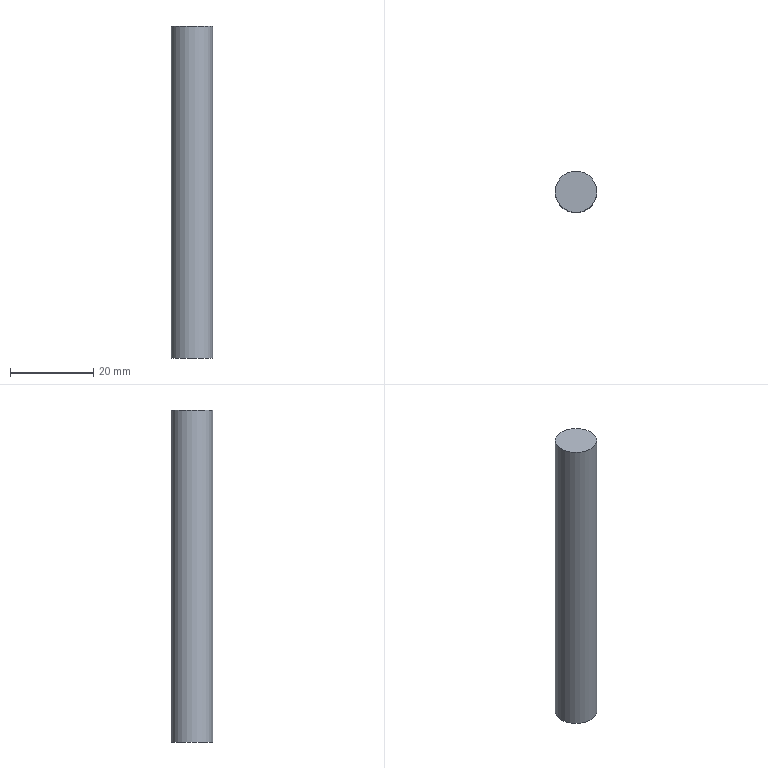Component | NX | FIXING_SCREW | 1 solid | 3 faces | box 10 x 10 x 80 mm | volume 6283 mm3 | plane 2 | cylinder 1 | commonest cylinder face diameters 10 x1
STEP:
#1=CARTESIAN_POINT('',(0.,0.,0.));
#2=DIRECTION('',(0.,0.,1.));
#3=DIRECTION('',(1.,0.,0.));
#4=AXIS2_PLACEMENT_3D('',#1,#2,#3);
#5=CARTESIAN_POINT('',(-5.,93.,139.));
#6=VERTEX_POINT('',#5);
#7=CARTESIAN_POINT('',(-0.,93.,139.));
#8=DIRECTION('',(0.,0.,-1.));
#9=DIRECTION('',(-1.,0.,0.));
#10=AXIS2_PLACEMENT_3D('',#7,#8,#9);
#11=CIRCLE('',#10,5.);
#12=CARTESIAN_POINT('',(-0.,93.,139.));
#13=DIRECTION('',(0.,0.,1.));
#14=DIRECTION('',(-1.,0.,0.));
#15=AXIS2_PLACEMENT_3D('',#12,#13,#14);
#16=PLANE('',#15);
#17=CARTESIAN_POINT('',(5.,0.));
#18=CARTESIAN_POINT('',(5.,-8.66));
#19=CARTESIAN_POINT('',(-2.5,-4.33));
#20=CARTESIAN_POINT('',(-10.,-0.));
#21=CARTESIAN_POINT('',(-2.5,4.33));
#22=CARTESIAN_POINT('',(5.,8.66));
#23=CARTESIAN_POINT('',(5.,0.));
#24=(BOUNDED_CURVE()B_SPLINE_CURVE(2,(#17,#18,#19,#20,#21,#22,#23),.UNSPECIFIED.,.T.,.F.)B_SPLINE_CURVE_WITH_KNOTS((1,2,2,2,2,1),(-2.094,0.,2.094,4.189,6.283,8.378),.UNSPECIFIED.)CURVE()GEOMETRIC_REPRESENTATION_ITEM()RATIONAL_B_SPLINE_CURVE((1.,0.5,1.,0.5,1.,0.5,1.))REPRESENTATION_ITEM(''));
#25=(GEOMETRIC_REPRESENTATION_CONTEXT(2)PARAMETRIC_REPRESENTATION_CONTEXT()REPRESENTATION_CONTEXT('',''));
#26=DEFINITIONAL_REPRESENTATION('',(#24),#25);
#27=PCURVE('',#16,#26);
#28=CARTESIAN_POINT('',(-0.,93.,59.));
#29=DIRECTION('',(0.,0.,1.));
#30=DIRECTION('',(-1.,0.,0.));
#31=AXIS2_PLACEMENT_3D('',#28,#29,#30);
#32=CYLINDRICAL_SURFACE('',#31,5.);
#33=CARTESIAN_POINT('',(6.283,80.));
#34=DIRECTION('',(-1.,0.));
#35=VECTOR('',#34,1.);
#36=LINE('',#33,#35);
#37=(GEOMETRIC_REPRESENTATION_CONTEXT(2)PARAMETRIC_REPRESENTATION_CONTEXT()REPRESENTATION_CONTEXT('',''));
#38=DEFINITIONAL_REPRESENTATION('',(#36),#37);
#39=PCURVE('',#32,#38);
#40=SURFACE_CURVE('',#11,(#27,#39),.PCURVE_S1.);
#41=EDGE_CURVE('',#6,#6,#40,.T.);
#42=ORIENTED_EDGE('',*,*,#41,.F.);
#43=EDGE_LOOP('',(#42));
#44=FACE_BOUND('',#43,.T.);
#45=ADVANCED_FACE('',(#44),#16,.T.);
#46=CARTESIAN_POINT('',(-5.,93.,59.));
#47=VERTEX_POINT('',#46);
#48=CARTESIAN_POINT('',(-0.,93.,59.));
#49=DIRECTION('',(0.,0.,1.));
#50=DIRECTION('',(-1.,0.,0.));
#51=AXIS2_PLACEMENT_3D('',#48,#49,#50);
#52=CIRCLE('',#51,5.);
#53=CARTESIAN_POINT('',(-0.,93.,59.));
#54=DIRECTION('',(0.,0.,-1.));
#55=DIRECTION('',(1.,0.,0.));
#56=AXIS2_PLACEMENT_3D('',#53,#54,#55);
#57=PLANE('',#56);
#58=CARTESIAN_POINT('',(-5.,0.));
#59=CARTESIAN_POINT('',(-5.,8.66));
#60=CARTESIAN_POINT('',(2.5,4.33));
#61=CARTESIAN_POINT('',(10.,0.));
#62=CARTESIAN_POINT('',(2.5,-4.33));
#63=CARTESIAN_POINT('',(-5.,-8.66));
#64=CARTESIAN_POINT('',(-5.,0.));
#65=(BOUNDED_CURVE()B_SPLINE_CURVE(2,(#58,#59,#60,#61,#62,#63,#64),.UNSPECIFIED.,.T.,.F.)B_SPLINE_CURVE_WITH_KNOTS((1,2,2,2,2,1),(-2.094,0.,2.094,4.189,6.283,8.378),.UNSPECIFIED.)CURVE()GEOMETRIC_REPRESENTATION_ITEM()RATIONAL_B_SPLINE_CURVE((1.,0.5,1.,0.5,1.,0.5,1.))REPRESENTATION_ITEM(''));
#66=(GEOMETRIC_REPRESENTATION_CONTEXT(2)PARAMETRIC_REPRESENTATION_CONTEXT()REPRESENTATION_CONTEXT('',''));
#67=DEFINITIONAL_REPRESENTATION('',(#65),#66);
#68=PCURVE('',#57,#67);
#69=CARTESIAN_POINT('',(0.,0.));
#70=DIRECTION('',(1.,0.));
#71=VECTOR('',#70,1.);
#72=LINE('',#69,#71);
#73=(GEOMETRIC_REPRESENTATION_CONTEXT(2)PARAMETRIC_REPRESENTATION_CONTEXT()REPRESENTATION_CONTEXT('',''));
#74=DEFINITIONAL_REPRESENTATION('',(#72),#73);
#75=PCURVE('',#32,#74);
#76=SURFACE_CURVE('',#52,(#68,#75),.PCURVE_S1.);
#77=EDGE_CURVE('',#47,#47,#76,.T.);
#78=ORIENTED_EDGE('',*,*,#77,.F.);
#79=EDGE_LOOP('',(#78));
#80=FACE_BOUND('',#79,.T.);
#81=ADVANCED_FACE('',(#80),#57,.T.);
#82=ORIENTED_EDGE('',*,*,#41,.T.);
#83=CARTESIAN_POINT('',(-5.,93.,59.));
#84=CARTESIAN_POINT('',(-5.,93.,139.));
#85=B_SPLINE_CURVE_WITH_KNOTS('',1,(#83,#84),.UNSPECIFIED.,.F.,.F.,(2,2),(0.,80.),.PIECEWISE_BEZIER_KNOTS.);
#86=CARTESIAN_POINT('',(0.,0.));
#87=DIRECTION('',(0.,1.));
#88=VECTOR('',#87,1.);
#89=LINE('',#86,#88);
#90=(GEOMETRIC_REPRESENTATION_CONTEXT(2)PARAMETRIC_REPRESENTATION_CONTEXT()REPRESENTATION_CONTEXT('',''));
#91=DEFINITIONAL_REPRESENTATION('',(#89),#90);
#92=PCURVE('',#32,#91);
#93=CARTESIAN_POINT('',(6.283,0.));
#94=DIRECTION('',(0.,1.));
#95=VECTOR('',#94,1.);
#96=LINE('',#93,#95);
#97=(GEOMETRIC_REPRESENTATION_CONTEXT(2)PARAMETRIC_REPRESENTATION_CONTEXT()REPRESENTATION_CONTEXT('',''));
#98=DEFINITIONAL_REPRESENTATION('',(#96),#97);
#99=PCURVE('',#32,#98);
#100=SEAM_CURVE('',#85,(#92,#99),.PCURVE_S1.);
#101=EDGE_CURVE('',#47,#6,#100,.T.);
#102=ORIENTED_EDGE('',*,*,#101,.F.);
#103=ORIENTED_EDGE('',*,*,#77,.T.);
#104=ORIENTED_EDGE('',*,*,#101,.T.);
#105=EDGE_LOOP('',(#82,#102,#103,#104));
#106=FACE_BOUND('',#105,.T.);
#107=ADVANCED_FACE('',(#106),#32,.T.);
#108=CLOSED_SHELL('',(#45,#81,#107));
#109=MANIFOLD_SOLID_BREP('',#108);
#110=(LENGTH_UNIT()NAMED_UNIT(*)SI_UNIT(.MILLI.,.METRE.));
#111=UNCERTAINTY_MEASURE_WITH_UNIT(LENGTH_MEASURE(0.00001),#110,'','');
#112=(NAMED_UNIT(*)PLANE_ANGLE_UNIT()SI_UNIT($,.RADIAN.));
#113=(NAMED_UNIT(*)SI_UNIT($,.STERADIAN.)SOLID_ANGLE_UNIT());
#114=(GEOMETRIC_REPRESENTATION_CONTEXT(3)GLOBAL_UNCERTAINTY_ASSIGNED_CONTEXT((#111))GLOBAL_UNIT_ASSIGNED_CONTEXT((#110,#112,#113))REPRESENTATION_CONTEXT('',''));
#115=ADVANCED_BREP_SHAPE_REPRESENTATION('',(#4,#109),#114);